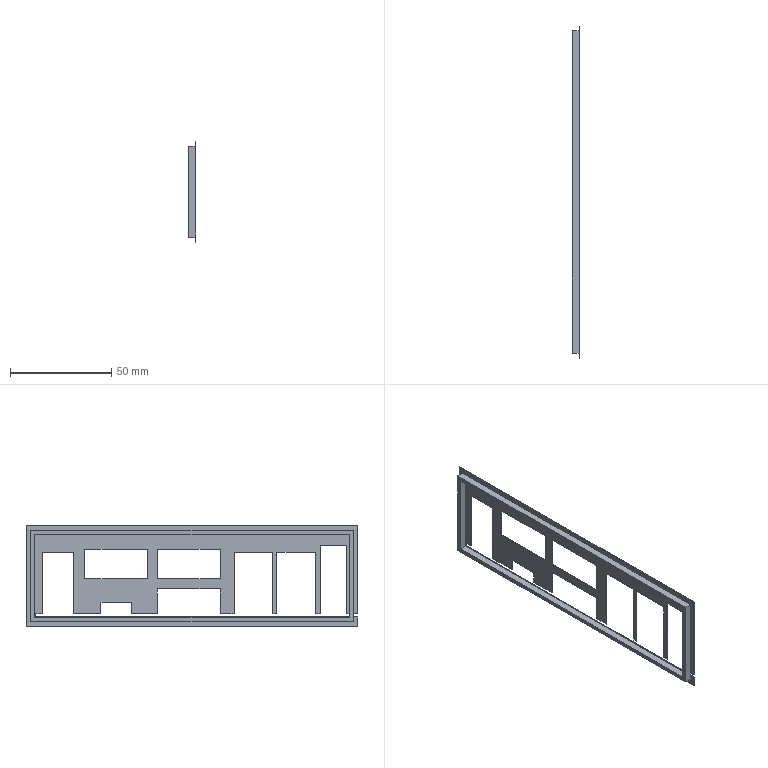Component | NX | BAFFLE | 1 solid | 53 faces | volume 3897 mm3 | plane 53